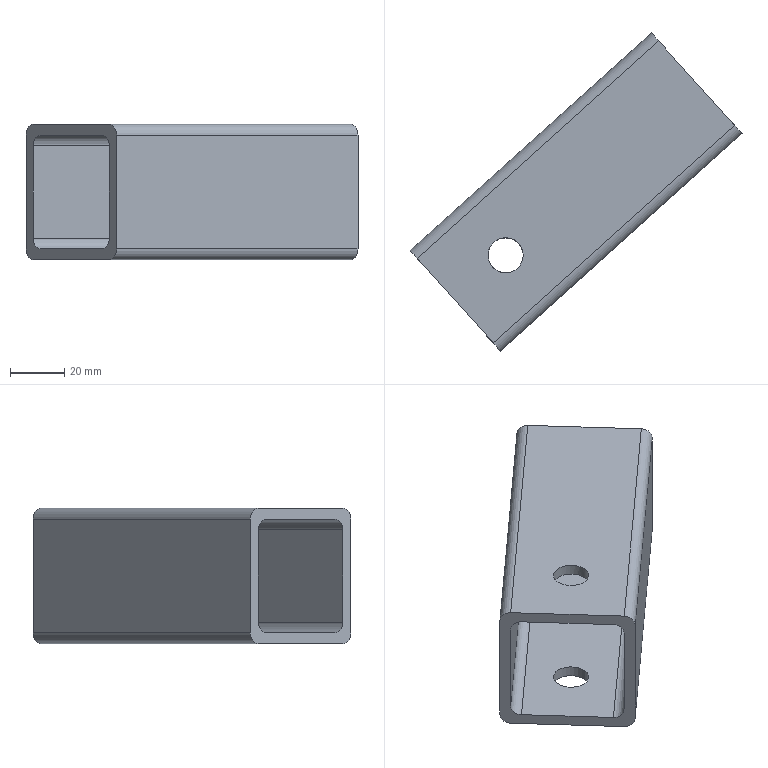Component | NX | ADJ_BRKT_CONN_BEAM | 1 solid | 20 faces | volume 87258 mm3 | plane 10 | cylinder 10 | commonest cylinder face diameters 8 x8 13 x2